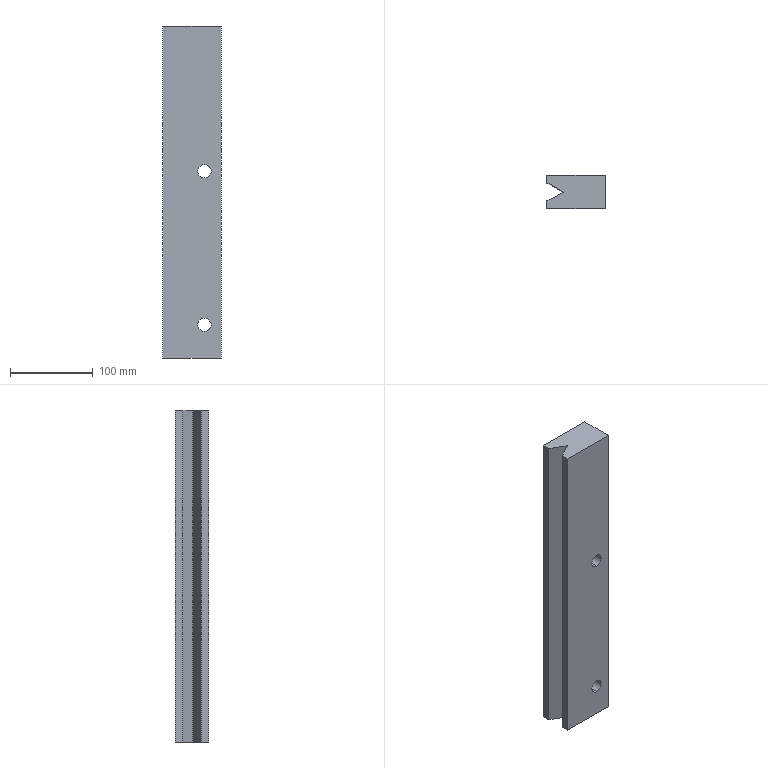Component | SolidWorks | GuidePlate-1 | 1 solid | 13 faces | box 70 x 40 x 400 mm | volume 1014695 mm3 | plane 9 | cylinder 4 | commonest cylinder face diameters 16 x4
build123d program:
from build123d import *

# Parameters (mm, degrees)
SKETCH1_W                  = 400
SKETCH1_H                  = 70
BOSS_EXTRUDE1_DEPTH        = 40
CUT_EXTRUDE1_DEPTH         = 411.268
DRAFT1_ANGLE               = 30.559
F_16_0_16_DIAMETER_HOLE1_D = 16


with BuildPart() as part:
    # Sketch1 → Boss-Extrude1 (new body)
    with BuildSketch(Plane(origin=(0, 0, 0), x_dir=(-1, 0, 0), z_dir=(0, 0, -1))):
        with Locations((-31.942, 46.975)):
            Rectangle(SKETCH1_W, SKETCH1_H)
    extrude(amount=-BOSS_EXTRUDE1_DEPTH)

    # Sketch2 → Cut-Extrude1 (cut, through all)
    with BuildSketch(Plane(origin=(231.942, 0, 0), x_dir=(0, 0, -1), z_dir=(1, 0, 0))):
        Polygon((-31.152, 81.975), (-8.848, 39.475), (-8.848, 81.975), align=None)
    extrude(amount=-CUT_EXTRUDE1_DEPTH, mode=Mode.SUBTRACT)

    # Draft1
    draft1_faces = [part.faces().sort_by_distance(p)[0] for p in [
        (31.942, 60.725, 8.848),
    ]]
    draft(draft1_faces, Plane(origin=(-168.058, 81.975, 40), x_dir=(1, 0, 0), z_dir=(0, 1, 0)), DRAFT1_ANGLE)

    # 16.0 _16_ Diameter Hole1 (through all)
    with Locations(Plane.XY.offset(40)):
        with Locations((-128.058, 31.975), (56.942, 31.975)):
            Hole(F_16_0_16_DIAMETER_HOLE1_D / 2)


solid = part.part

# Placed as in the assembly
solid = solid.moved(Location((-305.357, 957.548, 671.722), (90, 0, 90)))
STEP:
#1=CARTESIAN_POINT('',(-13.281,37.699,21.089));
#2=VERTEX_POINT('',#1);
#3=CARTESIAN_POINT('',(-13.281,37.699,21.719));
#4=VERTEX_POINT('',#3);
#5=CARTESIAN_POINT('',(-13.281,37.699,21.404));
#6=DIRECTION('',(0.,-1.,0.));
#7=DIRECTION('',(0.,0.,1.));
#8=AXIS2_PLACEMENT_3D('',#5,#6,#7);
#9=CIRCLE('',#8,0.315);
#10=EDGE_CURVE('',#2,#4,#9,.T.);
#11=ORIENTED_EDGE('',*,*,#10,.F.);
#12=CARTESIAN_POINT('',(-13.281,36.124,21.089));
#13=VERTEX_POINT('',#12);
#14=CARTESIAN_POINT('',(-13.281,36.124,21.089));
#15=DIRECTION('',(0.,-1.,0.));
#16=VECTOR('',#15,39.37);
#17=LINE('',#14,#16);
#18=EDGE_CURVE('',#2,#13,#17,.T.);
#19=ORIENTED_EDGE('',*,*,#18,.T.);
#20=CARTESIAN_POINT('',(-13.281,36.124,21.719));
#21=VERTEX_POINT('',#20);
#22=CARTESIAN_POINT('',(-13.281,36.124,21.404));
#23=DIRECTION('',(0.,-1.,0.));
#24=DIRECTION('',(0.,0.,1.));
#25=AXIS2_PLACEMENT_3D('',#22,#23,#24);
#26=CIRCLE('',#25,0.315);
#27=EDGE_CURVE('',#13,#21,#26,.T.);
#28=ORIENTED_EDGE('',*,*,#27,.T.);
#29=CARTESIAN_POINT('',(-13.281,36.124,21.719));
#30=DIRECTION('',(0.,-1.,0.));
#31=VECTOR('',#30,39.37);
#32=LINE('',#29,#31);
#33=EDGE_CURVE('',#4,#21,#32,.T.);
#34=ORIENTED_EDGE('',*,*,#33,.F.);
#35=EDGE_LOOP('',(#11,#19,#28,#34));
#36=FACE_OUTER_BOUND('',#35,.T.);
#37=CARTESIAN_POINT('',(-13.281,36.124,21.404));
#38=DIRECTION('',(0.,-1.,0.));
#39=DIRECTION('',(0.,0.,1.));
#40=AXIS2_PLACEMENT_3D('',#37,#38,#39);
#41=CYLINDRICAL_SURFACE('',#40,0.315);
#42=ADVANCED_FACE('',(#36),#41,.F.);
#43=CARTESIAN_POINT('',(-13.281,37.699,28.373));
#44=VERTEX_POINT('',#43);
#45=CARTESIAN_POINT('',(-13.281,37.699,29.002));
#46=VERTEX_POINT('',#45);
#47=CARTESIAN_POINT('',(-13.281,37.699,28.688));
#48=DIRECTION('',(0.,-1.,0.));
#49=DIRECTION('',(0.,0.,1.));
#50=AXIS2_PLACEMENT_3D('',#47,#48,#49);
#51=CIRCLE('',#50,0.315);
#52=EDGE_CURVE('',#44,#46,#51,.T.);
#53=ORIENTED_EDGE('',*,*,#52,.F.);
#54=CARTESIAN_POINT('',(-13.281,36.124,28.373));
#55=VERTEX_POINT('',#54);
#56=CARTESIAN_POINT('',(-13.281,36.124,28.373));
#57=DIRECTION('',(0.,-1.,0.));
#58=VECTOR('',#57,39.37);
#59=LINE('',#56,#58);
#60=EDGE_CURVE('',#44,#55,#59,.T.);
#61=ORIENTED_EDGE('',*,*,#60,.T.);
#62=CARTESIAN_POINT('',(-13.281,36.124,29.002));
#63=VERTEX_POINT('',#62);
#64=CARTESIAN_POINT('',(-13.281,36.124,28.688));
#65=DIRECTION('',(0.,-1.,0.));
#66=DIRECTION('',(0.,0.,1.));
#67=AXIS2_PLACEMENT_3D('',#64,#65,#66);
#68=CIRCLE('',#67,0.315);
#69=EDGE_CURVE('',#55,#63,#68,.T.);
#70=ORIENTED_EDGE('',*,*,#69,.T.);
#71=CARTESIAN_POINT('',(-13.281,36.124,29.002));
#72=DIRECTION('',(0.,-1.,0.));
#73=VECTOR('',#72,39.37);
#74=LINE('',#71,#73);
#75=EDGE_CURVE('',#46,#63,#74,.T.);
#76=ORIENTED_EDGE('',*,*,#75,.F.);
#77=EDGE_LOOP('',(#53,#61,#70,#76));
#78=FACE_OUTER_BOUND('',#77,.T.);
#79=CARTESIAN_POINT('',(-13.281,36.124,28.688));
#80=DIRECTION('',(0.,-1.,0.));
#81=DIRECTION('',(0.,0.,1.));
#82=AXIS2_PLACEMENT_3D('',#79,#80,#81);
#83=CYLINDRICAL_SURFACE('',#82,0.315);
#84=ADVANCED_FACE('',(#78),#83,.F.);
#85=CARTESIAN_POINT('',(-15.249,37.35,19.829));
#86=VERTEX_POINT('',#85);
#87=CARTESIAN_POINT('',(-15.249,37.35,35.577));
#88=VERTEX_POINT('',#87);
#89=CARTESIAN_POINT('',(-15.249,37.35,19.829));
#90=DIRECTION('',(0.,0.,1.));
#91=VECTOR('',#90,39.37);
#92=LINE('',#89,#91);
#93=EDGE_CURVE('',#86,#88,#92,.T.);
#94=ORIENTED_EDGE('',*,*,#93,.T.);
#95=CARTESIAN_POINT('',(-15.249,37.699,35.577));
#96=VERTEX_POINT('',#95);
#97=CARTESIAN_POINT('',(-15.249,36.124,35.577));
#98=DIRECTION('',(0.,1.,0.));
#99=VECTOR('',#98,39.37);
#100=LINE('',#97,#99);
#101=EDGE_CURVE('',#88,#96,#100,.T.);
#102=ORIENTED_EDGE('',*,*,#101,.T.);
#103=CARTESIAN_POINT('',(-15.249,37.699,19.829));
#104=VERTEX_POINT('',#103);
#105=CARTESIAN_POINT('',(-15.249,37.699,19.829));
#106=DIRECTION('',(0.,0.,1.));
#107=VECTOR('',#106,39.37);
#108=LINE('',#105,#107);
#109=EDGE_CURVE('',#104,#96,#108,.T.);
#110=ORIENTED_EDGE('',*,*,#109,.F.);
#111=CARTESIAN_POINT('',(-15.249,36.124,19.829));
#112=DIRECTION('',(0.,1.,0.));
#113=VECTOR('',#112,39.37);
#114=LINE('',#111,#113);
#115=EDGE_CURVE('',#86,#104,#114,.T.);
#116=ORIENTED_EDGE('',*,*,#115,.F.);
#117=EDGE_LOOP('',(#94,#102,#110,#116));
#118=FACE_OUTER_BOUND('',#117,.T.);
#119=CARTESIAN_POINT('',(-15.249,36.124,19.829));
#120=DIRECTION('',(-1.,0.,0.));
#121=DIRECTION('',(-0.,0.,-1.));
#122=AXIS2_PLACEMENT_3D('',#119,#120,#121);
#123=PLANE('',#122);
#124=ADVANCED_FACE('',(#118),#123,.T.);
#125=CARTESIAN_POINT('',(-14.462,36.886,35.577));
#126=VERTEX_POINT('',#125);
#127=CARTESIAN_POINT('',(-14.712,37.033,35.577));
#128=DIRECTION('',(-0.8611,0.5084,0.));
#129=VECTOR('',#128,39.37);
#130=LINE('',#127,#129);
#131=EDGE_CURVE('',#126,#88,#130,.T.);
#132=ORIENTED_EDGE('',*,*,#131,.F.);
#133=CARTESIAN_POINT('',(-15.249,36.472,35.577));
#134=VERTEX_POINT('',#133);
#135=CARTESIAN_POINT('',(-15.249,36.472,35.577));
#136=DIRECTION('',(0.8855,0.4647,0.));
#137=VECTOR('',#136,39.37);
#138=LINE('',#135,#137);
#139=EDGE_CURVE('',#134,#126,#138,.T.);
#140=ORIENTED_EDGE('',*,*,#139,.F.);
#141=CARTESIAN_POINT('',(-15.249,36.124,35.577));
#142=VERTEX_POINT('',#141);
#143=CARTESIAN_POINT('',(-15.249,36.124,35.577));
#144=DIRECTION('',(0.,1.,0.));
#145=VECTOR('',#144,39.37);
#146=LINE('',#143,#145);
#147=EDGE_CURVE('',#142,#134,#146,.T.);
#148=ORIENTED_EDGE('',*,*,#147,.F.);
#149=CARTESIAN_POINT('',(-12.493,36.124,35.577));
#150=VERTEX_POINT('',#149);
#151=CARTESIAN_POINT('',(-15.249,36.124,35.577));
#152=DIRECTION('',(1.,0.,0.));
#153=VECTOR('',#152,39.37);
#154=LINE('',#151,#153);
#155=EDGE_CURVE('',#142,#150,#154,.T.);
#156=ORIENTED_EDGE('',*,*,#155,.T.);
#157=CARTESIAN_POINT('',(-12.493,37.699,35.577));
#158=VERTEX_POINT('',#157);
#159=CARTESIAN_POINT('',(-12.493,36.124,35.577));
#160=DIRECTION('',(0.,1.,0.));
#161=VECTOR('',#160,39.37);
#162=LINE('',#159,#161);
#163=EDGE_CURVE('',#150,#158,#162,.T.);
#164=ORIENTED_EDGE('',*,*,#163,.T.);
#165=CARTESIAN_POINT('',(-15.249,37.699,35.577));
#166=DIRECTION('',(1.,0.,0.));
#167=VECTOR('',#166,39.37);
#168=LINE('',#165,#167);
#169=EDGE_CURVE('',#96,#158,#168,.T.);
#170=ORIENTED_EDGE('',*,*,#169,.F.);
#171=ORIENTED_EDGE('',*,*,#101,.F.);
#172=EDGE_LOOP('',(#132,#140,#148,#156,#164,#170,#171));
#173=FACE_OUTER_BOUND('',#172,.T.);
#174=CARTESIAN_POINT('',(-15.249,36.124,35.577));
#175=DIRECTION('',(0.,0.,1.));
#176=DIRECTION('',(0.,1.,0.));
#177=AXIS2_PLACEMENT_3D('',#174,#175,#176);
#178=PLANE('',#177);
#179=ADVANCED_FACE('',(#173),#178,.T.);
#180=CARTESIAN_POINT('',(-15.249,36.472,19.829));
#181=VERTEX_POINT('',#180);
#182=CARTESIAN_POINT('',(-15.249,36.472,19.829));
#183=DIRECTION('',(0.,0.,1.));
#184=VECTOR('',#183,39.37);
#185=LINE('',#182,#184);
#186=EDGE_CURVE('',#181,#134,#185,.T.);
#187=ORIENTED_EDGE('',*,*,#186,.F.);
#188=CARTESIAN_POINT('',(-15.249,36.124,19.829));
#189=VERTEX_POINT('',#188);
#190=CARTESIAN_POINT('',(-15.249,36.124,19.829));
#191=DIRECTION('',(0.,1.,0.));
#192=VECTOR('',#191,39.37);
#193=LINE('',#190,#192);
#194=EDGE_CURVE('',#189,#181,#193,.T.);
#195=ORIENTED_EDGE('',*,*,#194,.F.);
#196=CARTESIAN_POINT('',(-15.249,36.124,19.829));
#197=DIRECTION('',(0.,0.,1.));
#198=VECTOR('',#197,39.37);
#199=LINE('',#196,#198);
#200=EDGE_CURVE('',#189,#142,#199,.T.);
#201=ORIENTED_EDGE('',*,*,#200,.T.);
#202=ORIENTED_EDGE('',*,*,#147,.T.);
#203=EDGE_LOOP('',(#187,#195,#201,#202));
#204=FACE_OUTER_BOUND('',#203,.T.);
#205=CARTESIAN_POINT('',(-15.249,36.124,19.829));
#206=DIRECTION('',(-1.,0.,0.));
#207=DIRECTION('',(-0.,0.,-1.));
#208=AXIS2_PLACEMENT_3D('',#205,#206,#207);
#209=PLANE('',#208);
#210=ADVANCED_FACE('',(#204),#209,.T.);
#211=CARTESIAN_POINT('',(-14.462,36.886,19.829));
#212=VERTEX_POINT('',#211);
#213=CARTESIAN_POINT('',(-15.249,37.35,19.829));
#214=DIRECTION('',(-0.8611,0.5084,0.));
#215=VECTOR('',#214,39.37);
#216=LINE('',#213,#215);
#217=EDGE_CURVE('',#212,#86,#216,.T.);
#218=ORIENTED_EDGE('',*,*,#217,.T.);
#219=ORIENTED_EDGE('',*,*,#115,.T.);
#220=CARTESIAN_POINT('',(-12.493,37.699,19.829));
#221=VERTEX_POINT('',#220);
#222=CARTESIAN_POINT('',(-12.493,37.699,19.829));
#223=DIRECTION('',(-1.,0.,0.));
#224=VECTOR('',#223,39.37);
#225=LINE('',#222,#224);
#226=EDGE_CURVE('',#221,#104,#225,.T.);
#227=ORIENTED_EDGE('',*,*,#226,.F.);
#228=CARTESIAN_POINT('',(-12.493,36.124,19.829));
#229=VERTEX_POINT('',#228);
#230=CARTESIAN_POINT('',(-12.493,36.124,19.829));
#231=DIRECTION('',(0.,1.,0.));
#232=VECTOR('',#231,39.37);
#233=LINE('',#230,#232);
#234=EDGE_CURVE('',#229,#221,#233,.T.);
#235=ORIENTED_EDGE('',*,*,#234,.F.);
#236=CARTESIAN_POINT('',(-12.493,36.124,19.829));
#237=DIRECTION('',(-1.,0.,0.));
#238=VECTOR('',#237,39.37);
#239=LINE('',#236,#238);
#240=EDGE_CURVE('',#229,#189,#239,.T.);
#241=ORIENTED_EDGE('',*,*,#240,.T.);
#242=ORIENTED_EDGE('',*,*,#194,.T.);
#243=CARTESIAN_POINT('',(-15.249,36.472,19.829));
#244=DIRECTION('',(0.8855,0.4647,0.));
#245=VECTOR('',#244,39.37);
#246=LINE('',#243,#245);
#247=EDGE_CURVE('',#181,#212,#246,.T.);
#248=ORIENTED_EDGE('',*,*,#247,.T.);
#249=EDGE_LOOP('',(#218,#219,#227,#235,#241,#242,#248));
#250=FACE_OUTER_BOUND('',#249,.T.);
#251=CARTESIAN_POINT('',(-12.493,36.124,19.829));
#252=DIRECTION('',(0.,0.,-1.));
#253=DIRECTION('',(0.,-1.,0.));
#254=AXIS2_PLACEMENT_3D('',#251,#252,#253);
#255=PLANE('',#254);
#256=ADVANCED_FACE('',(#250),#255,.T.);
#257=CARTESIAN_POINT('',(-12.493,37.699,35.577));
#258=DIRECTION('',(0.,0.,-1.));
#259=VECTOR('',#258,39.37);
#260=LINE('',#257,#259);
#261=EDGE_CURVE('',#158,#221,#260,.T.);
#262=ORIENTED_EDGE('',*,*,#261,.F.);
#263=ORIENTED_EDGE('',*,*,#163,.F.);
#264=CARTESIAN_POINT('',(-12.493,36.124,35.577));
#265=DIRECTION('',(0.,0.,-1.));
#266=VECTOR('',#265,39.37);
#267=LINE('',#264,#266);
#268=EDGE_CURVE('',#150,#229,#267,.T.);
#269=ORIENTED_EDGE('',*,*,#268,.T.);
#270=ORIENTED_EDGE('',*,*,#234,.T.);
#271=EDGE_LOOP('',(#262,#263,#269,#270));
#272=FACE_OUTER_BOUND('',#271,.T.);
#273=CARTESIAN_POINT('',(-12.493,36.124,35.577));
#274=DIRECTION('',(1.,0.,0.));
#275=DIRECTION('',(-0.,0.,1.));
#276=AXIS2_PLACEMENT_3D('',#273,#274,#275);
#277=PLANE('',#276);
#278=ADVANCED_FACE('',(#272),#277,.T.);
#279=CARTESIAN_POINT('',(-13.281,36.124,21.404));
#280=DIRECTION('',(0.,-1.,0.));
#281=DIRECTION('',(0.,0.,1.));
#282=AXIS2_PLACEMENT_3D('',#279,#280,#281);
#283=CIRCLE('',#282,0.315);
#284=EDGE_CURVE('',#21,#13,#283,.T.);
#285=ORIENTED_EDGE('',*,*,#284,.F.);
#286=ORIENTED_EDGE('',*,*,#27,.F.);
#287=EDGE_LOOP('',(#285,#286));
#288=FACE_BOUND('',#287,.T.);
#289=CARTESIAN_POINT('',(-13.281,36.124,28.688));
#290=DIRECTION('',(0.,-1.,0.));
#291=DIRECTION('',(0.,0.,1.));
#292=AXIS2_PLACEMENT_3D('',#289,#290,#291);
#293=CIRCLE('',#292,0.315);
#294=EDGE_CURVE('',#63,#55,#293,.T.);
#295=ORIENTED_EDGE('',*,*,#294,.F.);
#296=ORIENTED_EDGE('',*,*,#69,.F.);
#297=EDGE_LOOP('',(#295,#296));
#298=FACE_BOUND('',#297,.T.);
#299=ORIENTED_EDGE('',*,*,#155,.F.);
#300=ORIENTED_EDGE('',*,*,#200,.F.);
#301=ORIENTED_EDGE('',*,*,#240,.F.);
#302=ORIENTED_EDGE('',*,*,#268,.F.);
#303=EDGE_LOOP('',(#299,#300,#301,#302));
#304=FACE_OUTER_BOUND('',#303,.T.);
#305=CARTESIAN_POINT('',(-12.022,36.124,26.446));
#306=DIRECTION('',(0.,1.,0.));
#307=DIRECTION('',(0.,0.,-1.));
#308=AXIS2_PLACEMENT_3D('',#305,#306,#307);
#309=PLANE('',#308);
#310=ADVANCED_FACE('',(#288,#298,#304),#309,.F.);
#311=CARTESIAN_POINT('',(-13.281,37.699,21.404));
#312=DIRECTION('',(0.,-1.,0.));
#313=DIRECTION('',(0.,0.,1.));
#314=AXIS2_PLACEMENT_3D('',#311,#312,#313);
#315=CIRCLE('',#314,0.315);
#316=EDGE_CURVE('',#4,#2,#315,.T.);
#317=ORIENTED_EDGE('',*,*,#316,.T.);
#318=ORIENTED_EDGE('',*,*,#10,.T.);
#319=EDGE_LOOP('',(#317,#318));
#320=FACE_BOUND('',#319,.T.);
#321=CARTESIAN_POINT('',(-13.281,37.699,28.688));
#322=DIRECTION('',(0.,-1.,0.));
#323=DIRECTION('',(0.,0.,1.));
#324=AXIS2_PLACEMENT_3D('',#321,#322,#323);
#325=CIRCLE('',#324,0.315);
#326=EDGE_CURVE('',#46,#44,#325,.T.);
#327=ORIENTED_EDGE('',*,*,#326,.T.);
#328=ORIENTED_EDGE('',*,*,#52,.T.);
#329=EDGE_LOOP('',(#327,#328));
#330=FACE_BOUND('',#329,.T.);
#331=ORIENTED_EDGE('',*,*,#169,.T.);
#332=ORIENTED_EDGE('',*,*,#261,.T.);
#333=ORIENTED_EDGE('',*,*,#226,.T.);
#334=ORIENTED_EDGE('',*,*,#109,.T.);
#335=EDGE_LOOP('',(#331,#332,#333,#334));
#336=FACE_OUTER_BOUND('',#335,.T.);
#337=CARTESIAN_POINT('',(-12.022,37.699,26.446));
#338=DIRECTION('',(0.,1.,0.));
#339=DIRECTION('',(0.,0.,-1.));
#340=AXIS2_PLACEMENT_3D('',#337,#338,#339);
#341=PLANE('',#340);
#342=ADVANCED_FACE('',(#320,#330,#336),#341,.T.);
#343=ORIENTED_EDGE('',*,*,#131,.T.);
#344=ORIENTED_EDGE('',*,*,#93,.F.);
#345=ORIENTED_EDGE('',*,*,#217,.F.);
#346=CARTESIAN_POINT('',(-14.462,36.886,19.829));
#347=DIRECTION('',(0.,0.,1.));
#348=VECTOR('',#347,39.37);
#349=LINE('',#346,#348);
#350=EDGE_CURVE('',#212,#126,#349,.T.);
#351=ORIENTED_EDGE('',*,*,#350,.T.);
#352=EDGE_LOOP('',(#343,#344,#345,#351));
#353=FACE_OUTER_BOUND('',#352,.T.);
#354=CARTESIAN_POINT('',(-15.249,37.35,19.829));
#355=DIRECTION('',(-0.5084,-0.8611,0.));
#356=DIRECTION('',(0.8611,-0.5084,0.));
#357=AXIS2_PLACEMENT_3D('',#354,#355,#356);
#358=PLANE('',#357);
#359=ADVANCED_FACE('',(#353),#358,.T.);
#360=ORIENTED_EDGE('',*,*,#139,.T.);
#361=ORIENTED_EDGE('',*,*,#350,.F.);
#362=ORIENTED_EDGE('',*,*,#247,.F.);
#363=ORIENTED_EDGE('',*,*,#186,.T.);
#364=EDGE_LOOP('',(#360,#361,#362,#363));
#365=FACE_OUTER_BOUND('',#364,.T.);
#366=CARTESIAN_POINT('',(-15.249,36.472,19.829));
#367=DIRECTION('',(0.4647,-0.8855,0.));
#368=DIRECTION('',(0.8855,0.4647,0.));
#369=AXIS2_PLACEMENT_3D('',#366,#367,#368);
#370=PLANE('',#369);
#371=ADVANCED_FACE('',(#365),#370,.F.);
#372=ORIENTED_EDGE('',*,*,#60,.F.);
#373=ORIENTED_EDGE('',*,*,#326,.F.);
#374=ORIENTED_EDGE('',*,*,#75,.T.);
#375=ORIENTED_EDGE('',*,*,#294,.T.);
#376=EDGE_LOOP('',(#372,#373,#374,#375));
#377=FACE_OUTER_BOUND('',#376,.T.);
#378=CARTESIAN_POINT('',(-13.281,36.124,28.688));
#379=DIRECTION('',(0.,-1.,0.));
#380=DIRECTION('',(0.,0.,1.));
#381=AXIS2_PLACEMENT_3D('',#378,#379,#380);
#382=CYLINDRICAL_SURFACE('',#381,0.315);
#383=ADVANCED_FACE('',(#377),#382,.F.);
#384=ORIENTED_EDGE('',*,*,#18,.F.);
#385=ORIENTED_EDGE('',*,*,#316,.F.);
#386=ORIENTED_EDGE('',*,*,#33,.T.);
#387=ORIENTED_EDGE('',*,*,#284,.T.);
#388=EDGE_LOOP('',(#384,#385,#386,#387));
#389=FACE_OUTER_BOUND('',#388,.T.);
#390=CARTESIAN_POINT('',(-13.281,36.124,21.404));
#391=DIRECTION('',(0.,-1.,0.));
#392=DIRECTION('',(0.,0.,1.));
#393=AXIS2_PLACEMENT_3D('',#390,#391,#392);
#394=CYLINDRICAL_SURFACE('',#393,0.315);
#395=ADVANCED_FACE('',(#389),#394,.F.);
#396=CLOSED_SHELL('',(#42,#84,#124,#179,#210,#256,#278,#310,#342,#359,#371,#383,#395));
#397=MANIFOLD_SOLID_BREP('',#396);
#398=CARTESIAN_POINT('',(0.,0.,0.));
#399=DIRECTION('',(0.,0.,1.));
#400=DIRECTION('',(1.,0.,0.));
#401=AXIS2_PLACEMENT_3D('',#398,#399,#400);
#402=(LENGTH_UNIT()NAMED_UNIT(*)SI_UNIT($,.METRE.));
#403=LENGTH_MEASURE_WITH_UNIT(LENGTH_MEASURE(0.0254),#402);
#404=DIMENSIONAL_EXPONENTS(1.,0.,0.,0.,0.,0.,0.);
#405=(CONVERSION_BASED_UNIT('',#403)LENGTH_UNIT()NAMED_UNIT(#404));
#406=UNCERTAINTY_MEASURE_WITH_UNIT(LENGTH_MEASURE(0.00001),#405,'','');
#407=(NAMED_UNIT(*)PLANE_ANGLE_UNIT()SI_UNIT($,.RADIAN.));
#408=(NAMED_UNIT(*)SI_UNIT($,.STERADIAN.)SOLID_ANGLE_UNIT());
#409=(GEOMETRIC_REPRESENTATION_CONTEXT(3)GLOBAL_UNCERTAINTY_ASSIGNED_CONTEXT((#406))GLOBAL_UNIT_ASSIGNED_CONTEXT((#405,#407,#408))REPRESENTATION_CONTEXT('',''));
#410=ADVANCED_BREP_SHAPE_REPRESENTATION('',(#397,#401),#409);
#411=COLOUR_RGB('',0.7922,0.8196,0.9333);
#412=FILL_AREA_STYLE_COLOUR('',#411);
#413=FILL_AREA_STYLE('',(#412));
#414=SURFACE_STYLE_FILL_AREA(#413);
#415=SURFACE_SIDE_STYLE('',(#414));
#416=SURFACE_STYLE_USAGE(.BOTH.,#415);
#417=PRESENTATION_STYLE_ASSIGNMENT((#416));
#418=STYLED_ITEM('',(#417),#397);
#419=(LENGTH_UNIT()NAMED_UNIT(*)SI_UNIT($,.METRE.));
#420=LENGTH_MEASURE_WITH_UNIT(LENGTH_MEASURE(0.0254),#419);
#421=DIMENSIONAL_EXPONENTS(1.,0.,0.,0.,0.,0.,0.);
#422=(CONVERSION_BASED_UNIT('',#420)LENGTH_UNIT()NAMED_UNIT(#421));
#423=UNCERTAINTY_MEASURE_WITH_UNIT(LENGTH_MEASURE(0.00001),#422,'','');
#424=(NAMED_UNIT(*)PLANE_ANGLE_UNIT()SI_UNIT($,.RADIAN.));
#425=(NAMED_UNIT(*)SI_UNIT($,.STERADIAN.)SOLID_ANGLE_UNIT());
#426=(GEOMETRIC_REPRESENTATION_CONTEXT(3)GLOBAL_UNCERTAINTY_ASSIGNED_CONTEXT((#423))GLOBAL_UNIT_ASSIGNED_CONTEXT((#422,#424,#425))REPRESENTATION_CONTEXT('',''));
#427=MECHANICAL_DESIGN_GEOMETRIC_PRESENTATION_REPRESENTATION('',(#418),#426);
#428=PRESENTATION_LAYER_ASSIGNMENT('','',(#418));